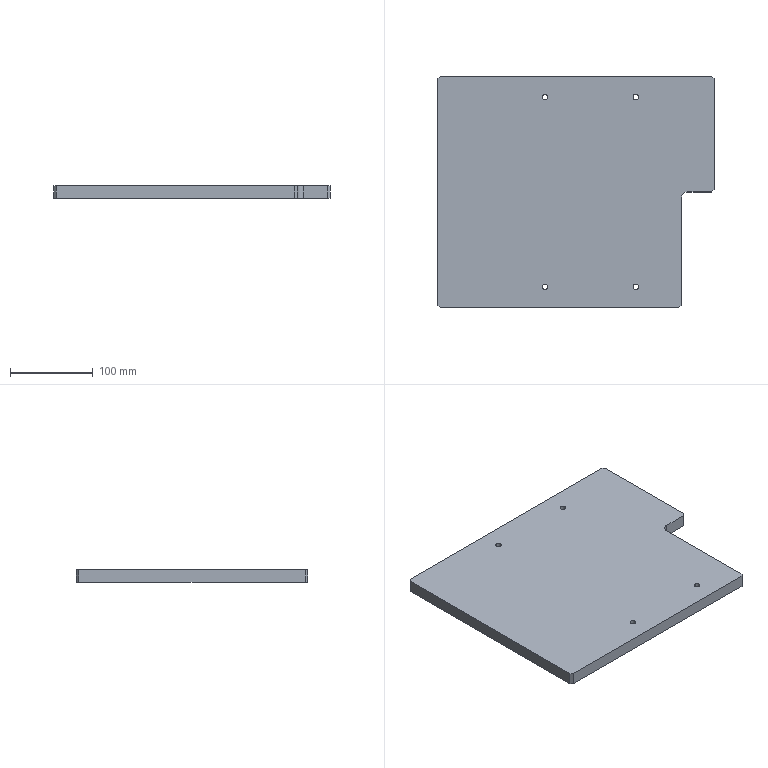Component | SolidWorks | STE21014.01-45-1 | 1 solid | 22 faces | box 335 x 280 x 15 mm | volume 1320690 mm3 | plane 13 | cylinder 9 | commonest cylinder face diameters 6.8 x8 16 x1 | material Q235
build123d program:
from build123d import *

# Parameters (mm, degrees)
SKETCH1_W           = 335
SKETCH1_H           = 280
BOSS_EXTRUDE1_DEPTH = 15
SKETCH4_W           = 40
SKETCH4_H           = 140
CUT_EXTRUDE1_DEPTH  = 219.818
M8_TAPPED_HOLE1_D   = 6.8
FILLET1_R           = 8
CHAMFER2_SIZE       = 3


with BuildPart() as part:
    # Sketch1 → Boss-Extrude1 (new body)
    with BuildSketch(Plane(origin=(0, 0, 0), x_dir=(1, 0, 0), z_dir=(0, 1, 0))):
        Rectangle(SKETCH1_W, SKETCH1_H)
    extrude(amount=BOSS_EXTRUDE1_DEPTH)

    # Sketch4 → Cut-Extrude1 (cut, through all)
    with BuildSketch(Plane(origin=(0, 15, 0), x_dir=(1, 0, 0), z_dir=(0, 1, 0))):
        with Locations((147.5, 70)):
            Rectangle(SKETCH4_W, SKETCH4_H)
    extrude(amount=-CUT_EXTRUDE1_DEPTH, mode=Mode.SUBTRACT)

    # M8 Tapped Hole1 (through all)
    with Locations(Plane(origin=(0, 15, 0), x_dir=(1, 0, 0), z_dir=(0, 1, 0))):
        with Locations((-37.5, -115), (72.5, -115), (-37.5, 115), (72.5, 115)):
            Hole(M8_TAPPED_HOLE1_D / 2)

    # Fillet1
    fillet1_edges = [part.edges().sort_by_distance(p)[0] for p in [
        (127.5, 7.5, 0),
    ]]
    fillet(fillet1_edges, radius=FILLET1_R)

    # Chamfer2
    chamfer2_edges = [part.edges().sort_by_distance(p)[0] for p in [
        (127.5, 7.5, -140),
        (167.5, 7.5, 0),
        (-167.5, 7.5, -140),
        (167.5, 7.5, 140),
        (-167.5, 7.5, 140),
    ]]
    chamfer(chamfer2_edges, length=CHAMFER2_SIZE)


solid = part.part

# Placed as in the assembly
solid = solid.moved(Location((137.5, 523.5, -90), (-90, 0, 0)))
STEP:
#1=COLOUR_RGB('',0.7922,0.8196,0.9333);
#2=FILL_AREA_STYLE_COLOUR('',#1);
#3=FILL_AREA_STYLE('',(#2));
#4=SURFACE_STYLE_FILL_AREA(#3);
#5=SURFACE_SIDE_STYLE('',(#4));
#6=SURFACE_STYLE_USAGE(.BOTH.,#5);
#7=PRESENTATION_STYLE_ASSIGNMENT((#6));
#8=CARTESIAN_POINT('',(3.937,25.004,-3.543));
#9=VERTEX_POINT('',#8);
#10=CARTESIAN_POINT('',(3.937,25.272,-3.543));
#11=VERTEX_POINT('',#10);
#12=CARTESIAN_POINT('',(3.937,25.138,-3.543));
#13=DIRECTION('',(0.,0.,-1.));
#14=DIRECTION('',(0.,1.,0.));
#15=AXIS2_PLACEMENT_3D('',#12,#13,#14);
#16=CIRCLE('',#15,0.1339);
#17=EDGE_CURVE('',#9,#11,#16,.T.);
#18=ORIENTED_EDGE('',*,*,#17,.F.);
#19=CARTESIAN_POINT('',(3.937,25.004,-4.134));
#20=VERTEX_POINT('',#19);
#21=CARTESIAN_POINT('',(3.937,25.004,-4.134));
#22=DIRECTION('',(0.,0.,-1.));
#23=VECTOR('',#22,39.37);
#24=LINE('',#21,#23);
#25=EDGE_CURVE('',#9,#20,#24,.T.);
#26=ORIENTED_EDGE('',*,*,#25,.T.);
#27=CARTESIAN_POINT('',(3.937,25.272,-4.134));
#28=VERTEX_POINT('',#27);
#29=CARTESIAN_POINT('',(3.937,25.138,-4.134));
#30=DIRECTION('',(0.,0.,-1.));
#31=DIRECTION('',(0.,1.,0.));
#32=AXIS2_PLACEMENT_3D('',#29,#30,#31);
#33=CIRCLE('',#32,0.1339);
#34=EDGE_CURVE('',#20,#28,#33,.T.);
#35=ORIENTED_EDGE('',*,*,#34,.T.);
#36=CARTESIAN_POINT('',(3.937,25.272,-4.134));
#37=DIRECTION('',(0.,0.,-1.));
#38=VECTOR('',#37,39.37);
#39=LINE('',#36,#38);
#40=EDGE_CURVE('',#11,#28,#39,.T.);
#41=ORIENTED_EDGE('',*,*,#40,.F.);
#42=EDGE_LOOP('',(#18,#26,#35,#41));
#43=FACE_OUTER_BOUND('',#42,.T.);
#44=CARTESIAN_POINT('',(3.937,25.138,-4.134));
#45=DIRECTION('',(0.,0.,-1.));
#46=DIRECTION('',(0.,1.,0.));
#47=AXIS2_PLACEMENT_3D('',#44,#45,#46);
#48=CYLINDRICAL_SURFACE('',#47,0.1339);
#49=ADVANCED_FACE('',(#43),#48,.F.);
#50=CARTESIAN_POINT('',(8.268,25.004,-3.543));
#51=VERTEX_POINT('',#50);
#52=CARTESIAN_POINT('',(8.268,25.272,-3.543));
#53=VERTEX_POINT('',#52);
#54=CARTESIAN_POINT('',(8.268,25.138,-3.543));
#55=DIRECTION('',(0.,0.,-1.));
#56=DIRECTION('',(0.,1.,0.));
#57=AXIS2_PLACEMENT_3D('',#54,#55,#56);
#58=CIRCLE('',#57,0.1339);
#59=EDGE_CURVE('',#51,#53,#58,.T.);
#60=ORIENTED_EDGE('',*,*,#59,.F.);
#61=CARTESIAN_POINT('',(8.268,25.004,-4.134));
#62=VERTEX_POINT('',#61);
#63=CARTESIAN_POINT('',(8.268,25.004,-4.134));
#64=DIRECTION('',(0.,0.,-1.));
#65=VECTOR('',#64,39.37);
#66=LINE('',#63,#65);
#67=EDGE_CURVE('',#51,#62,#66,.T.);
#68=ORIENTED_EDGE('',*,*,#67,.T.);
#69=CARTESIAN_POINT('',(8.268,25.272,-4.134));
#70=VERTEX_POINT('',#69);
#71=CARTESIAN_POINT('',(8.268,25.138,-4.134));
#72=DIRECTION('',(0.,0.,-1.));
#73=DIRECTION('',(0.,1.,0.));
#74=AXIS2_PLACEMENT_3D('',#71,#72,#73);
#75=CIRCLE('',#74,0.1339);
#76=EDGE_CURVE('',#62,#70,#75,.T.);
#77=ORIENTED_EDGE('',*,*,#76,.T.);
#78=CARTESIAN_POINT('',(8.268,25.272,-4.134));
#79=DIRECTION('',(0.,0.,-1.));
#80=VECTOR('',#79,39.37);
#81=LINE('',#78,#80);
#82=EDGE_CURVE('',#53,#70,#81,.T.);
#83=ORIENTED_EDGE('',*,*,#82,.F.);
#84=EDGE_LOOP('',(#60,#68,#77,#83));
#85=FACE_OUTER_BOUND('',#84,.T.);
#86=CARTESIAN_POINT('',(8.268,25.138,-4.134));
#87=DIRECTION('',(0.,0.,-1.));
#88=DIRECTION('',(0.,1.,0.));
#89=AXIS2_PLACEMENT_3D('',#86,#87,#88);
#90=CYLINDRICAL_SURFACE('',#89,0.1339);
#91=ADVANCED_FACE('',(#85),#90,.F.);
#92=CARTESIAN_POINT('',(3.937,15.949,-3.543));
#93=VERTEX_POINT('',#92);
#94=CARTESIAN_POINT('',(3.937,16.217,-3.543));
#95=VERTEX_POINT('',#94);
#96=CARTESIAN_POINT('',(3.937,16.083,-3.543));
#97=DIRECTION('',(0.,0.,-1.));
#98=DIRECTION('',(0.,1.,0.));
#99=AXIS2_PLACEMENT_3D('',#96,#97,#98);
#100=CIRCLE('',#99,0.1339);
#101=EDGE_CURVE('',#93,#95,#100,.T.);
#102=ORIENTED_EDGE('',*,*,#101,.F.);
#103=CARTESIAN_POINT('',(3.937,15.949,-4.134));
#104=VERTEX_POINT('',#103);
#105=CARTESIAN_POINT('',(3.937,15.949,-4.134));
#106=DIRECTION('',(0.,0.,-1.));
#107=VECTOR('',#106,39.37);
#108=LINE('',#105,#107);
#109=EDGE_CURVE('',#93,#104,#108,.T.);
#110=ORIENTED_EDGE('',*,*,#109,.T.);
#111=CARTESIAN_POINT('',(3.937,16.217,-4.134));
#112=VERTEX_POINT('',#111);
#113=CARTESIAN_POINT('',(3.937,16.083,-4.134));
#114=DIRECTION('',(0.,0.,-1.));
#115=DIRECTION('',(0.,1.,0.));
#116=AXIS2_PLACEMENT_3D('',#113,#114,#115);
#117=CIRCLE('',#116,0.1339);
#118=EDGE_CURVE('',#104,#112,#117,.T.);
#119=ORIENTED_EDGE('',*,*,#118,.T.);
#120=CARTESIAN_POINT('',(3.937,16.217,-4.134));
#121=DIRECTION('',(0.,0.,-1.));
#122=VECTOR('',#121,39.37);
#123=LINE('',#120,#122);
#124=EDGE_CURVE('',#95,#112,#123,.T.);
#125=ORIENTED_EDGE('',*,*,#124,.F.);
#126=EDGE_LOOP('',(#102,#110,#119,#125));
#127=FACE_OUTER_BOUND('',#126,.T.);
#128=CARTESIAN_POINT('',(3.937,16.083,-4.134));
#129=DIRECTION('',(0.,0.,-1.));
#130=DIRECTION('',(0.,1.,0.));
#131=AXIS2_PLACEMENT_3D('',#128,#129,#130);
#132=CYLINDRICAL_SURFACE('',#131,0.1339);
#133=ADVANCED_FACE('',(#127),#132,.F.);
#134=CARTESIAN_POINT('',(8.268,15.949,-3.543));
#135=VERTEX_POINT('',#134);
#136=CARTESIAN_POINT('',(8.268,16.217,-3.543));
#137=VERTEX_POINT('',#136);
#138=CARTESIAN_POINT('',(8.268,16.083,-3.543));
#139=DIRECTION('',(0.,0.,-1.));
#140=DIRECTION('',(0.,1.,0.));
#141=AXIS2_PLACEMENT_3D('',#138,#139,#140);
#142=CIRCLE('',#141,0.1339);
#143=EDGE_CURVE('',#135,#137,#142,.T.);
#144=ORIENTED_EDGE('',*,*,#143,.F.);
#145=CARTESIAN_POINT('',(8.268,15.949,-4.134));
#146=VERTEX_POINT('',#145);
#147=CARTESIAN_POINT('',(8.268,15.949,-4.134));
#148=DIRECTION('',(0.,0.,-1.));
#149=VECTOR('',#148,39.37);
#150=LINE('',#147,#149);
#151=EDGE_CURVE('',#135,#146,#150,.T.);
#152=ORIENTED_EDGE('',*,*,#151,.T.);
#153=CARTESIAN_POINT('',(8.268,16.217,-4.134));
#154=VERTEX_POINT('',#153);
#155=CARTESIAN_POINT('',(8.268,16.083,-4.134));
#156=DIRECTION('',(0.,0.,-1.));
#157=DIRECTION('',(0.,1.,0.));
#158=AXIS2_PLACEMENT_3D('',#155,#156,#157);
#159=CIRCLE('',#158,0.1339);
#160=EDGE_CURVE('',#146,#154,#159,.T.);
#161=ORIENTED_EDGE('',*,*,#160,.T.);
#162=CARTESIAN_POINT('',(8.268,16.217,-4.134));
#163=DIRECTION('',(0.,0.,-1.));
#164=VECTOR('',#163,39.37);
#165=LINE('',#162,#164);
#166=EDGE_CURVE('',#137,#154,#165,.T.);
#167=ORIENTED_EDGE('',*,*,#166,.F.);
#168=EDGE_LOOP('',(#144,#152,#161,#167));
#169=FACE_OUTER_BOUND('',#168,.T.);
#170=CARTESIAN_POINT('',(8.268,16.083,-4.134));
#171=DIRECTION('',(0.,0.,-1.));
#172=DIRECTION('',(0.,1.,0.));
#173=AXIS2_PLACEMENT_3D('',#170,#171,#172);
#174=CYLINDRICAL_SURFACE('',#173,0.1339);
#175=ADVANCED_FACE('',(#169),#174,.F.);
#176=CARTESIAN_POINT('',(-1.181,15.217,-4.134));
#177=VERTEX_POINT('',#176);
#178=CARTESIAN_POINT('',(-1.181,26.004,-4.134));
#179=VERTEX_POINT('',#178);
#180=CARTESIAN_POINT('',(-1.181,26.122,-4.134));
#181=DIRECTION('',(0.,1.,0.));
#182=VECTOR('',#181,39.37);
#183=LINE('',#180,#182);
#184=EDGE_CURVE('',#177,#179,#183,.T.);
#185=ORIENTED_EDGE('',*,*,#184,.F.);
#186=CARTESIAN_POINT('',(-1.181,15.217,-3.543));
#187=VERTEX_POINT('',#186);
#188=CARTESIAN_POINT('',(-1.181,15.217,-4.134));
#189=DIRECTION('',(-0.,-0.,1.));
#190=VECTOR('',#189,39.37);
#191=LINE('',#188,#190);
#192=EDGE_CURVE('',#177,#187,#191,.T.);
#193=ORIENTED_EDGE('',*,*,#192,.T.);
#194=CARTESIAN_POINT('',(-1.181,26.004,-3.543));
#195=VERTEX_POINT('',#194);
#196=CARTESIAN_POINT('',(-1.181,26.122,-3.543));
#197=DIRECTION('',(0.,1.,0.));
#198=VECTOR('',#197,39.37);
#199=LINE('',#196,#198);
#200=EDGE_CURVE('',#187,#195,#199,.T.);
#201=ORIENTED_EDGE('',*,*,#200,.T.);
#202=CARTESIAN_POINT('',(-1.181,26.004,-4.134));
#203=DIRECTION('',(0.,0.,-1.));
#204=VECTOR('',#203,39.37);
#205=LINE('',#202,#204);
#206=EDGE_CURVE('',#195,#179,#205,.T.);
#207=ORIENTED_EDGE('',*,*,#206,.T.);
#208=EDGE_LOOP('',(#185,#193,#201,#207));
#209=FACE_OUTER_BOUND('',#208,.T.);
#210=CARTESIAN_POINT('',(-1.181,26.122,-4.134));
#211=DIRECTION('',(1.,0.,-0.));
#212=DIRECTION('',(-0.,-1.,-0.));
#213=AXIS2_PLACEMENT_3D('',#210,#211,#212);
#214=PLANE('',#213);
#215=ADVANCED_FACE('',(#209),#214,.F.);
#216=CARTESIAN_POINT('',(-1.063,26.122,-4.134));
#217=VERTEX_POINT('',#216);
#218=CARTESIAN_POINT('',(11.89,26.122,-4.134));
#219=VERTEX_POINT('',#218);
#220=CARTESIAN_POINT('',(12.008,26.122,-4.134));
#221=DIRECTION('',(1.,-0.,-0.));
#222=VECTOR('',#221,39.37);
#223=LINE('',#220,#222);
#224=EDGE_CURVE('',#217,#219,#223,.T.);
#225=ORIENTED_EDGE('',*,*,#224,.F.);
#226=CARTESIAN_POINT('',(-1.063,26.122,-3.543));
#227=VERTEX_POINT('',#226);
#228=CARTESIAN_POINT('',(-1.063,26.122,-4.134));
#229=DIRECTION('',(-0.,-0.,1.));
#230=VECTOR('',#229,39.37);
#231=LINE('',#228,#230);
#232=EDGE_CURVE('',#217,#227,#231,.T.);
#233=ORIENTED_EDGE('',*,*,#232,.T.);
#234=CARTESIAN_POINT('',(11.89,26.122,-3.543));
#235=VERTEX_POINT('',#234);
#236=CARTESIAN_POINT('',(12.008,26.122,-3.543));
#237=DIRECTION('',(1.,-0.,-0.));
#238=VECTOR('',#237,39.37);
#239=LINE('',#236,#238);
#240=EDGE_CURVE('',#227,#235,#239,.T.);
#241=ORIENTED_EDGE('',*,*,#240,.T.);
#242=CARTESIAN_POINT('',(11.89,26.122,-4.134));
#243=DIRECTION('',(0.,0.,-1.));
#244=VECTOR('',#243,39.37);
#245=LINE('',#242,#244);
#246=EDGE_CURVE('',#235,#219,#245,.T.);
#247=ORIENTED_EDGE('',*,*,#246,.T.);
#248=EDGE_LOOP('',(#225,#233,#241,#247));
#249=FACE_OUTER_BOUND('',#248,.T.);
#250=CARTESIAN_POINT('',(12.008,26.122,-4.134));
#251=DIRECTION('',(-0.,-1.,-0.));
#252=DIRECTION('',(-1.,0.,0.));
#253=AXIS2_PLACEMENT_3D('',#250,#251,#252);
#254=PLANE('',#253);
#255=ADVANCED_FACE('',(#249),#254,.F.);
#256=CARTESIAN_POINT('',(12.008,26.004,-3.543));
#257=VERTEX_POINT('',#256);
#258=CARTESIAN_POINT('',(12.008,20.728,-3.543));
#259=VERTEX_POINT('',#258);
#260=CARTESIAN_POINT('',(12.008,26.122,-3.543));
#261=DIRECTION('',(-0.,-1.,-0.));
#262=VECTOR('',#261,39.37);
#263=LINE('',#260,#262);
#264=EDGE_CURVE('',#257,#259,#263,.T.);
#265=ORIENTED_EDGE('',*,*,#264,.T.);
#266=CARTESIAN_POINT('',(12.008,20.728,-4.134));
#267=VERTEX_POINT('',#266);
#268=CARTESIAN_POINT('',(12.008,20.728,-4.134));
#269=DIRECTION('',(0.,0.,-1.));
#270=VECTOR('',#269,39.37);
#271=LINE('',#268,#270);
#272=EDGE_CURVE('',#259,#267,#271,.T.);
#273=ORIENTED_EDGE('',*,*,#272,.T.);
#274=CARTESIAN_POINT('',(12.008,26.004,-4.134));
#275=VERTEX_POINT('',#274);
#276=CARTESIAN_POINT('',(12.008,26.122,-4.134));
#277=DIRECTION('',(-0.,-1.,-0.));
#278=VECTOR('',#277,39.37);
#279=LINE('',#276,#278);
#280=EDGE_CURVE('',#275,#267,#279,.T.);
#281=ORIENTED_EDGE('',*,*,#280,.F.);
#282=CARTESIAN_POINT('',(12.008,26.004,-4.134));
#283=DIRECTION('',(-0.,-0.,1.));
#284=VECTOR('',#283,39.37);
#285=LINE('',#282,#284);
#286=EDGE_CURVE('',#275,#257,#285,.T.);
#287=ORIENTED_EDGE('',*,*,#286,.T.);
#288=EDGE_LOOP('',(#265,#273,#281,#287));
#289=FACE_OUTER_BOUND('',#288,.T.);
#290=CARTESIAN_POINT('',(12.008,26.122,-4.134));
#291=DIRECTION('',(-1.,-0.,0.));
#292=DIRECTION('',(0.,1.,0.));
#293=AXIS2_PLACEMENT_3D('',#290,#291,#292);
#294=PLANE('',#293);
#295=ADVANCED_FACE('',(#289),#294,.F.);
#296=CARTESIAN_POINT('',(10.315,15.098,-3.543));
#297=VERTEX_POINT('',#296);
#298=CARTESIAN_POINT('',(-1.063,15.098,-3.543));
#299=VERTEX_POINT('',#298);
#300=CARTESIAN_POINT('',(12.008,15.098,-3.543));
#301=DIRECTION('',(-1.,0.,0.));
#302=VECTOR('',#301,39.37);
#303=LINE('',#300,#302);
#304=EDGE_CURVE('',#297,#299,#303,.T.);
#305=ORIENTED_EDGE('',*,*,#304,.T.);
#306=CARTESIAN_POINT('',(-1.063,15.098,-4.134));
#307=VERTEX_POINT('',#306);
#308=CARTESIAN_POINT('',(-1.063,15.098,-4.134));
#309=DIRECTION('',(0.,0.,-1.));
#310=VECTOR('',#309,39.37);
#311=LINE('',#308,#310);
#312=EDGE_CURVE('',#299,#307,#311,.T.);
#313=ORIENTED_EDGE('',*,*,#312,.T.);
#314=CARTESIAN_POINT('',(10.315,15.098,-4.134));
#315=VERTEX_POINT('',#314);
#316=CARTESIAN_POINT('',(12.008,15.098,-4.134));
#317=DIRECTION('',(-1.,0.,0.));
#318=VECTOR('',#317,39.37);
#319=LINE('',#316,#318);
#320=EDGE_CURVE('',#315,#307,#319,.T.);
#321=ORIENTED_EDGE('',*,*,#320,.F.);
#322=CARTESIAN_POINT('',(10.315,15.098,-4.134));
#323=DIRECTION('',(-0.,-0.,1.));
#324=VECTOR('',#323,39.37);
#325=LINE('',#322,#324);
#326=EDGE_CURVE('',#315,#297,#325,.T.);
#327=ORIENTED_EDGE('',*,*,#326,.T.);
#328=EDGE_LOOP('',(#305,#313,#321,#327));
#329=FACE_OUTER_BOUND('',#328,.T.);
#330=CARTESIAN_POINT('',(12.008,15.098,-4.134));
#331=DIRECTION('',(0.,1.,0.));
#332=DIRECTION('',(1.,-0.,-0.));
#333=AXIS2_PLACEMENT_3D('',#330,#331,#332);
#334=PLANE('',#333);
#335=ADVANCED_FACE('',(#329),#334,.F.);
#336=CARTESIAN_POINT('',(3.937,25.138,-4.134));
#337=DIRECTION('',(0.,0.,-1.));
#338=DIRECTION('',(0.,1.,0.));
#339=AXIS2_PLACEMENT_3D('',#336,#337,#338);
#340=CIRCLE('',#339,0.1339);
#341=EDGE_CURVE('',#28,#20,#340,.T.);
#342=ORIENTED_EDGE('',*,*,#341,.F.);
#343=ORIENTED_EDGE('',*,*,#34,.F.);
#344=EDGE_LOOP('',(#342,#343));
#345=FACE_BOUND('',#344,.T.);
#346=CARTESIAN_POINT('',(8.268,25.138,-4.134));
#347=DIRECTION('',(0.,0.,-1.));
#348=DIRECTION('',(0.,1.,0.));
#349=AXIS2_PLACEMENT_3D('',#346,#347,#348);
#350=CIRCLE('',#349,0.1339);
#351=EDGE_CURVE('',#70,#62,#350,.T.);
#352=ORIENTED_EDGE('',*,*,#351,.F.);
#353=ORIENTED_EDGE('',*,*,#76,.F.);
#354=EDGE_LOOP('',(#352,#353));
#355=FACE_BOUND('',#354,.T.);
#356=CARTESIAN_POINT('',(3.937,16.083,-4.134));
#357=DIRECTION('',(0.,0.,-1.));
#358=DIRECTION('',(0.,1.,0.));
#359=AXIS2_PLACEMENT_3D('',#356,#357,#358);
#360=CIRCLE('',#359,0.1339);
#361=EDGE_CURVE('',#112,#104,#360,.T.);
#362=ORIENTED_EDGE('',*,*,#361,.F.);
#363=ORIENTED_EDGE('',*,*,#118,.F.);
#364=EDGE_LOOP('',(#362,#363));
#365=FACE_BOUND('',#364,.T.);
#366=CARTESIAN_POINT('',(8.268,16.083,-4.134));
#367=DIRECTION('',(0.,0.,-1.));
#368=DIRECTION('',(0.,1.,0.));
#369=AXIS2_PLACEMENT_3D('',#366,#367,#368);
#370=CIRCLE('',#369,0.1339);
#371=EDGE_CURVE('',#154,#146,#370,.T.);
#372=ORIENTED_EDGE('',*,*,#371,.F.);
#373=ORIENTED_EDGE('',*,*,#160,.F.);
#374=EDGE_LOOP('',(#372,#373));
#375=FACE_BOUND('',#374,.T.);
#376=ORIENTED_EDGE('',*,*,#280,.T.);
#377=CARTESIAN_POINT('',(11.89,20.61,-4.134));
#378=VERTEX_POINT('',#377);
#379=CARTESIAN_POINT('',(8.652,17.372,-4.134));
#380=DIRECTION('',(-0.7071,-0.7071,0.));
#381=VECTOR('',#380,39.37);
#382=LINE('',#379,#381);
#383=EDGE_CURVE('',#267,#378,#382,.T.);
#384=ORIENTED_EDGE('',*,*,#383,.T.);
#385=CARTESIAN_POINT('',(10.748,20.61,-4.134));
#386=VERTEX_POINT('',#385);
#387=CARTESIAN_POINT('',(10.433,20.61,-4.134));
#388=DIRECTION('',(1.,-0.,-0.));
#389=VECTOR('',#388,39.37);
#390=LINE('',#387,#389);
#391=EDGE_CURVE('',#386,#378,#390,.T.);
#392=ORIENTED_EDGE('',*,*,#391,.F.);
#393=CARTESIAN_POINT('',(10.433,20.295,-4.134));
#394=VERTEX_POINT('',#393);
#395=CARTESIAN_POINT('',(10.748,20.295,-4.134));
#396=DIRECTION('',(-0.,-0.,1.));
#397=DIRECTION('',(0.,1.,0.));
#398=AXIS2_PLACEMENT_3D('',#395,#396,#397);
#399=CIRCLE('',#398,0.315);
#400=EDGE_CURVE('',#386,#394,#399,.T.);
#401=ORIENTED_EDGE('',*,*,#400,.T.);
#402=CARTESIAN_POINT('',(10.433,15.217,-4.134));
#403=VERTEX_POINT('',#402);
#404=CARTESIAN_POINT('',(10.433,20.61,-4.134));
#405=DIRECTION('',(0.,1.,0.));
#406=VECTOR('',#405,39.37);
#407=LINE('',#404,#406);
#408=EDGE_CURVE('',#403,#394,#407,.T.);
#409=ORIENTED_EDGE('',*,*,#408,.F.);
#410=CARTESIAN_POINT('',(10.62,15.404,-4.134));
#411=DIRECTION('',(-0.7071,-0.7071,0.));
#412=VECTOR('',#411,39.37);
#413=LINE('',#410,#412);
#414=EDGE_CURVE('',#403,#315,#413,.T.);
#415=ORIENTED_EDGE('',*,*,#414,.T.);
#416=ORIENTED_EDGE('',*,*,#320,.T.);
#417=CARTESIAN_POINT('',(-0.5807,14.616,-4.134));
#418=DIRECTION('',(-0.7071,0.7071,0.));
#419=VECTOR('',#418,39.37);
#420=LINE('',#417,#419);
#421=EDGE_CURVE('',#307,#177,#420,.T.);
#422=ORIENTED_EDGE('',*,*,#421,.T.);
#423=ORIENTED_EDGE('',*,*,#184,.T.);
#424=CARTESIAN_POINT('',(-0.5807,26.604,-4.134));
#425=DIRECTION('',(0.7071,0.7071,-0.));
#426=VECTOR('',#425,39.37);
#427=LINE('',#424,#426);
#428=EDGE_CURVE('',#179,#217,#427,.T.);
#429=ORIENTED_EDGE('',*,*,#428,.T.);
#430=ORIENTED_EDGE('',*,*,#224,.T.);
#431=CARTESIAN_POINT('',(11.407,26.604,-4.134));
#432=DIRECTION('',(0.7071,-0.7071,-0.));
#433=VECTOR('',#432,39.37);
#434=LINE('',#431,#433);
#435=EDGE_CURVE('',#219,#275,#434,.T.);
#436=ORIENTED_EDGE('',*,*,#435,.T.);
#437=EDGE_LOOP('',(#376,#384,#392,#401,#409,#415,#416,#422,#423,#429,#430,#436));
#438=FACE_OUTER_BOUND('',#437,.T.);
#439=CARTESIAN_POINT('',(5.413,20.61,-4.134));
#440=DIRECTION('',(0.,0.,-1.));
#441=DIRECTION('',(0.,1.,0.));
#442=AXIS2_PLACEMENT_3D('',#439,#440,#441);
#443=PLANE('',#442);
#444=ADVANCED_FACE('',(#345,#355,#365,#375,#438),#443,.T.);
#445=CARTESIAN_POINT('',(3.937,25.138,-3.543));
#446=DIRECTION('',(0.,0.,-1.));
#447=DIRECTION('',(0.,1.,0.));
#448=AXIS2_PLACEMENT_3D('',#445,#446,#447);
#449=CIRCLE('',#448,0.1339);
#450=EDGE_CURVE('',#11,#9,#449,.T.);
#451=ORIENTED_EDGE('',*,*,#450,.T.);
#452=ORIENTED_EDGE('',*,*,#17,.T.);
#453=EDGE_LOOP('',(#451,#452));
#454=FACE_BOUND('',#453,.T.);
#455=CARTESIAN_POINT('',(8.268,25.138,-3.543));
#456=DIRECTION('',(0.,0.,-1.));
#457=DIRECTION('',(0.,1.,0.));
#458=AXIS2_PLACEMENT_3D('',#455,#456,#457);
#459=CIRCLE('',#458,0.1339);
#460=EDGE_CURVE('',#53,#51,#459,.T.);
#461=ORIENTED_EDGE('',*,*,#460,.T.);
#462=ORIENTED_EDGE('',*,*,#59,.T.);
#463=EDGE_LOOP('',(#461,#462));
#464=FACE_BOUND('',#463,.T.);
#465=CARTESIAN_POINT('',(3.937,16.083,-3.543));
#466=DIRECTION('',(0.,0.,-1.));
#467=DIRECTION('',(0.,1.,0.));
#468=AXIS2_PLACEMENT_3D('',#465,#466,#467);
#469=CIRCLE('',#468,0.1339);
#470=EDGE_CURVE('',#95,#93,#469,.T.);
#471=ORIENTED_EDGE('',*,*,#470,.T.);
#472=ORIENTED_EDGE('',*,*,#101,.T.);
#473=EDGE_LOOP('',(#471,#472));
#474=FACE_BOUND('',#473,.T.);
#475=CARTESIAN_POINT('',(8.268,16.083,-3.543));
#476=DIRECTION('',(0.,0.,-1.));
#477=DIRECTION('',(0.,1.,0.));
#478=AXIS2_PLACEMENT_3D('',#475,#476,#477);
#479=CIRCLE('',#478,0.1339);
#480=EDGE_CURVE('',#137,#135,#479,.T.);
#481=ORIENTED_EDGE('',*,*,#480,.T.);
#482=ORIENTED_EDGE('',*,*,#143,.T.);
#483=EDGE_LOOP('',(#481,#482));
#484=FACE_BOUND('',#483,.T.);
#485=CARTESIAN_POINT('',(10.748,20.61,-3.543));
#486=VERTEX_POINT('',#485);
#487=CARTESIAN_POINT('',(11.89,20.61,-3.543));
#488=VERTEX_POINT('',#487);
#489=CARTESIAN_POINT('',(10.433,20.61,-3.543));
#490=DIRECTION('',(1.,-0.,-0.));
#491=VECTOR('',#490,39.37);
#492=LINE('',#489,#491);
#493=EDGE_CURVE('',#486,#488,#492,.T.);
#494=ORIENTED_EDGE('',*,*,#493,.T.);
#495=CARTESIAN_POINT('',(12.008,20.728,-3.543));
#496=DIRECTION('',(0.7071,0.7071,-0.));
#497=VECTOR('',#496,39.37);
#498=LINE('',#495,#497);
#499=EDGE_CURVE('',#488,#259,#498,.T.);
#500=ORIENTED_EDGE('',*,*,#499,.T.);
#501=ORIENTED_EDGE('',*,*,#264,.F.);
#502=CARTESIAN_POINT('',(12.008,26.004,-3.543));
#503=DIRECTION('',(-0.7071,0.7071,0.));
#504=VECTOR('',#503,39.37);
#505=LINE('',#502,#504);
#506=EDGE_CURVE('',#257,#235,#505,.T.);
#507=ORIENTED_EDGE('',*,*,#506,.T.);
#508=ORIENTED_EDGE('',*,*,#240,.F.);
#509=CARTESIAN_POINT('',(-1.063,26.122,-3.543));
#510=DIRECTION('',(-0.7071,-0.7071,0.));
#511=VECTOR('',#510,39.37);
#512=LINE('',#509,#511);
#513=EDGE_CURVE('',#227,#195,#512,.T.);
#514=ORIENTED_EDGE('',*,*,#513,.T.);
#515=ORIENTED_EDGE('',*,*,#200,.F.);
#516=CARTESIAN_POINT('',(-1.181,15.217,-3.543));
#517=DIRECTION('',(0.7071,-0.7071,-0.));
#518=VECTOR('',#517,39.37);
#519=LINE('',#516,#518);
#520=EDGE_CURVE('',#187,#299,#519,.T.);
#521=ORIENTED_EDGE('',*,*,#520,.T.);
#522=ORIENTED_EDGE('',*,*,#304,.F.);
#523=CARTESIAN_POINT('',(10.433,15.217,-3.543));
#524=VERTEX_POINT('',#523);
#525=CARTESIAN_POINT('',(10.433,15.217,-3.543));
#526=DIRECTION('',(0.7071,0.7071,-0.));
#527=VECTOR('',#526,39.37);
#528=LINE('',#525,#527);
#529=EDGE_CURVE('',#297,#524,#528,.T.);
#530=ORIENTED_EDGE('',*,*,#529,.T.);
#531=CARTESIAN_POINT('',(10.433,20.295,-3.543));
#532=VERTEX_POINT('',#531);
#533=CARTESIAN_POINT('',(10.433,20.61,-3.543));
#534=DIRECTION('',(0.,1.,0.));
#535=VECTOR('',#534,39.37);
#536=LINE('',#533,#535);
#537=EDGE_CURVE('',#524,#532,#536,.T.);
#538=ORIENTED_EDGE('',*,*,#537,.T.);
#539=CARTESIAN_POINT('',(10.748,20.295,-3.543));
#540=DIRECTION('',(0.,0.,-1.));
#541=DIRECTION('',(0.,1.,0.));
#542=AXIS2_PLACEMENT_3D('',#539,#540,#541);
#543=CIRCLE('',#542,0.315);
#544=EDGE_CURVE('',#532,#486,#543,.T.);
#545=ORIENTED_EDGE('',*,*,#544,.T.);
#546=EDGE_LOOP('',(#494,#500,#501,#507,#508,#514,#515,#521,#522,#530,#538,#545));
#547=FACE_OUTER_BOUND('',#546,.T.);
#548=CARTESIAN_POINT('',(5.413,20.61,-3.543));
#549=DIRECTION('',(0.,0.,-1.));
#550=DIRECTION('',(0.,1.,0.));
#551=AXIS2_PLACEMENT_3D('',#548,#549,#550);
#552=PLANE('',#551);
#553=ADVANCED_FACE('',(#454,#464,#474,#484,#547),#552,.F.);
#554=ORIENTED_EDGE('',*,*,#537,.F.);
#555=CARTESIAN_POINT('',(10.433,15.217,-3.543));
#556=DIRECTION('',(0.,0.,-1.));
#557=VECTOR('',#556,39.37);
#558=LINE('',#555,#557);
#559=EDGE_CURVE('',#524,#403,#558,.T.);
#560=ORIENTED_EDGE('',*,*,#559,.T.);
#561=ORIENTED_EDGE('',*,*,#408,.T.);
#562=CARTESIAN_POINT('',(10.433,20.295,-3.543));
#563=DIRECTION('',(-0.,-0.,1.));
#564=VECTOR('',#563,39.37);
#565=LINE('',#562,#564);
#566=EDGE_CURVE('',#394,#532,#565,.T.);
#567=ORIENTED_EDGE('',*,*,#566,.T.);
#568=EDGE_LOOP('',(#554,#560,#561,#567));
#569=FACE_OUTER_BOUND('',#568,.T.);
#570=CARTESIAN_POINT('',(10.433,20.61,-3.543));
#571=DIRECTION('',(-1.,-0.,0.));
#572=DIRECTION('',(0.,1.,0.));
#573=AXIS2_PLACEMENT_3D('',#570,#571,#572);
#574=PLANE('',#573);
#575=ADVANCED_FACE('',(#569),#574,.F.);
#576=ORIENTED_EDGE('',*,*,#391,.T.);
#577=CARTESIAN_POINT('',(11.89,20.61,-3.543));
#578=DIRECTION('',(-0.,-0.,1.));
#579=VECTOR('',#578,39.37);
#580=LINE('',#577,#579);
#581=EDGE_CURVE('',#378,#488,#580,.T.);
#582=ORIENTED_EDGE('',*,*,#581,.T.);
#583=ORIENTED_EDGE('',*,*,#493,.F.);
#584=CARTESIAN_POINT('',(10.748,20.61,-4.134));
#585=DIRECTION('',(0.,0.,-1.));
#586=VECTOR('',#585,39.37);
#587=LINE('',#584,#586);
#588=EDGE_CURVE('',#486,#386,#587,.T.);
#589=ORIENTED_EDGE('',*,*,#588,.T.);
#590=EDGE_LOOP('',(#576,#582,#583,#589));
#591=FACE_OUTER_BOUND('',#590,.T.);
#592=CARTESIAN_POINT('',(10.433,20.61,-3.543));
#593=DIRECTION('',(0.,1.,0.));
#594=DIRECTION('',(1.,-0.,-0.));
#595=AXIS2_PLACEMENT_3D('',#592,#593,#594);
#596=PLANE('',#595);
#597=ADVANCED_FACE('',(#591),#596,.F.);
#598=ORIENTED_EDGE('',*,*,#151,.F.);
#599=ORIENTED_EDGE('',*,*,#480,.F.);
#600=ORIENTED_EDGE('',*,*,#166,.T.);
#601=ORIENTED_EDGE('',*,*,#371,.T.);
#602=EDGE_LOOP('',(#598,#599,#600,#601));
#603=FACE_OUTER_BOUND('',#602,.T.);
#604=CARTESIAN_POINT('',(8.268,16.083,-4.134));
#605=DIRECTION('',(0.,0.,-1.));
#606=DIRECTION('',(0.,1.,0.));
#607=AXIS2_PLACEMENT_3D('',#604,#605,#606);
#608=CYLINDRICAL_SURFACE('',#607,0.1339);
#609=ADVANCED_FACE('',(#603),#608,.F.);
#610=ORIENTED_EDGE('',*,*,#109,.F.);
#611=ORIENTED_EDGE('',*,*,#470,.F.);
#612=ORIENTED_EDGE('',*,*,#124,.T.);
#613=ORIENTED_EDGE('',*,*,#361,.T.);
#614=EDGE_LOOP('',(#610,#611,#612,#613));
#615=FACE_OUTER_BOUND('',#614,.T.);
#616=CARTESIAN_POINT('',(3.937,16.083,-4.134));
#617=DIRECTION('',(0.,0.,-1.));
#618=DIRECTION('',(0.,1.,0.));
#619=AXIS2_PLACEMENT_3D('',#616,#617,#618);
#620=CYLINDRICAL_SURFACE('',#619,0.1339);
#621=ADVANCED_FACE('',(#615),#620,.F.);
#622=ORIENTED_EDGE('',*,*,#67,.F.);
#623=ORIENTED_EDGE('',*,*,#460,.F.);
#624=ORIENTED_EDGE('',*,*,#82,.T.);
#625=ORIENTED_EDGE('',*,*,#351,.T.);
#626=EDGE_LOOP('',(#622,#623,#624,#625));
#627=FACE_OUTER_BOUND('',#626,.T.);
#628=CARTESIAN_POINT('',(8.268,25.138,-4.134));
#629=DIRECTION('',(0.,0.,-1.));
#630=DIRECTION('',(0.,1.,0.));
#631=AXIS2_PLACEMENT_3D('',#628,#629,#630);
#632=CYLINDRICAL_SURFACE('',#631,0.1339);
#633=ADVANCED_FACE('',(#627),#632,.F.);
#634=ORIENTED_EDGE('',*,*,#25,.F.);
#635=ORIENTED_EDGE('',*,*,#450,.F.);
#636=ORIENTED_EDGE('',*,*,#40,.T.);
#637=ORIENTED_EDGE('',*,*,#341,.T.);
#638=EDGE_LOOP('',(#634,#635,#636,#637));
#639=FACE_OUTER_BOUND('',#638,.T.);
#640=CARTESIAN_POINT('',(3.937,25.138,-4.134));
#641=DIRECTION('',(0.,0.,-1.));
#642=DIRECTION('',(0.,1.,0.));
#643=AXIS2_PLACEMENT_3D('',#640,#641,#642);
#644=CYLINDRICAL_SURFACE('',#643,0.1339);
#645=ADVANCED_FACE('',(#639),#644,.F.);
#646=ORIENTED_EDGE('',*,*,#544,.F.);
#647=ORIENTED_EDGE('',*,*,#566,.F.);
#648=ORIENTED_EDGE('',*,*,#400,.F.);
#649=ORIENTED_EDGE('',*,*,#588,.F.);
#650=EDGE_LOOP('',(#646,#647,#648,#649));
#651=FACE_OUTER_BOUND('',#650,.T.);
#652=CARTESIAN_POINT('',(10.748,20.295,-3.543));
#653=DIRECTION('',(-0.,-0.,1.));
#654=DIRECTION('',(0.,-1.,0.));
#655=AXIS2_PLACEMENT_3D('',#652,#653,#654);
#656=CYLINDRICAL_SURFACE('',#655,0.315);
#657=ADVANCED_FACE('',(#651),#656,.F.);
#658=ORIENTED_EDGE('',*,*,#499,.F.);
#659=ORIENTED_EDGE('',*,*,#581,.F.);
#660=ORIENTED_EDGE('',*,*,#383,.F.);
#661=ORIENTED_EDGE('',*,*,#272,.F.);
#662=EDGE_LOOP('',(#658,#659,#660,#661));
#663=FACE_OUTER_BOUND('',#662,.T.);
#664=CARTESIAN_POINT('',(12.008,20.728,-4.134));
#665=DIRECTION('',(-0.7071,0.7071,0.));
#666=DIRECTION('',(0.,0.,-1.));
#667=AXIS2_PLACEMENT_3D('',#664,#665,#666);
#668=PLANE('',#667);
#669=ADVANCED_FACE('',(#663),#668,.F.);
#670=ORIENTED_EDGE('',*,*,#421,.F.);
#671=ORIENTED_EDGE('',*,*,#312,.F.);
#672=ORIENTED_EDGE('',*,*,#520,.F.);
#673=ORIENTED_EDGE('',*,*,#192,.F.);
#674=EDGE_LOOP('',(#670,#671,#672,#673));
#675=FACE_OUTER_BOUND('',#674,.T.);
#676=CARTESIAN_POINT('',(-1.181,15.217,-4.134));
#677=DIRECTION('',(0.7071,0.7071,0.));
#678=DIRECTION('',(-0.,-0.,1.));
#679=AXIS2_PLACEMENT_3D('',#676,#677,#678);
#680=PLANE('',#679);
#681=ADVANCED_FACE('',(#675),#680,.F.);
#682=ORIENTED_EDGE('',*,*,#428,.F.);
#683=ORIENTED_EDGE('',*,*,#206,.F.);
#684=ORIENTED_EDGE('',*,*,#513,.F.);
#685=ORIENTED_EDGE('',*,*,#232,.F.);
#686=EDGE_LOOP('',(#682,#683,#684,#685));
#687=FACE_OUTER_BOUND('',#686,.T.);
#688=CARTESIAN_POINT('',(-1.063,26.122,-4.134));
#689=DIRECTION('',(0.7071,-0.7071,-0.));
#690=DIRECTION('',(-0.,-0.,1.));
#691=AXIS2_PLACEMENT_3D('',#688,#689,#690);
#692=PLANE('',#691);
#693=ADVANCED_FACE('',(#687),#692,.F.);
#694=ORIENTED_EDGE('',*,*,#435,.F.);
#695=ORIENTED_EDGE('',*,*,#246,.F.);
#696=ORIENTED_EDGE('',*,*,#506,.F.);
#697=ORIENTED_EDGE('',*,*,#286,.F.);
#698=EDGE_LOOP('',(#694,#695,#696,#697));
#699=FACE_OUTER_BOUND('',#698,.T.);
#700=CARTESIAN_POINT('',(12.008,26.004,-4.134));
#701=DIRECTION('',(-0.7071,-0.7071,-0.));
#702=DIRECTION('',(-0.,-0.,1.));
#703=AXIS2_PLACEMENT_3D('',#700,#701,#702);
#704=PLANE('',#703);
#705=ADVANCED_FACE('',(#699),#704,.F.);
#706=ORIENTED_EDGE('',*,*,#529,.F.);
#707=ORIENTED_EDGE('',*,*,#326,.F.);
#708=ORIENTED_EDGE('',*,*,#414,.F.);
#709=ORIENTED_EDGE('',*,*,#559,.F.);
#710=EDGE_LOOP('',(#706,#707,#708,#709));
#711=FACE_OUTER_BOUND('',#710,.T.);
#712=CARTESIAN_POINT('',(10.433,15.217,-3.543));
#713=DIRECTION('',(-0.7071,0.7071,0.));
#714=DIRECTION('',(0.,0.,-1.));
#715=AXIS2_PLACEMENT_3D('',#712,#713,#714);
#716=PLANE('',#715);
#717=ADVANCED_FACE('',(#711),#716,.F.);
#718=CLOSED_SHELL('',(#49,#91,#133,#175,#215,#255,#295,#335,#444,#553,#575,#597,#609,#621,#633,#645,#657,#669,#681,#693,#705,#717));
#719=MANIFOLD_SOLID_BREP('',#718);
#720=STYLED_ITEM('',(#7),#719);
#721=(LENGTH_UNIT()NAMED_UNIT(*)SI_UNIT($,.METRE.));
#722=LENGTH_MEASURE_WITH_UNIT(LENGTH_MEASURE(0.0254),#721);
#723=DIMENSIONAL_EXPONENTS(1.,0.,0.,0.,0.,0.,0.);
#724=(CONVERSION_BASED_UNIT('',#722)LENGTH_UNIT()NAMED_UNIT(#723));
#725=UNCERTAINTY_MEASURE_WITH_UNIT(LENGTH_MEASURE(0.00001),#724,'','');
#726=(NAMED_UNIT(*)PLANE_ANGLE_UNIT()SI_UNIT($,.RADIAN.));
#727=(NAMED_UNIT(*)SI_UNIT($,.STERADIAN.)SOLID_ANGLE_UNIT());
#728=(GEOMETRIC_REPRESENTATION_CONTEXT(3)GLOBAL_UNCERTAINTY_ASSIGNED_CONTEXT((#725))GLOBAL_UNIT_ASSIGNED_CONTEXT((#724,#726,#727))REPRESENTATION_CONTEXT('',''));
#729=MECHANICAL_DESIGN_GEOMETRIC_PRESENTATION_REPRESENTATION('',(#720),#728);
#730=CARTESIAN_POINT('',(0.,0.,0.));
#731=DIRECTION('',(0.,0.,1.));
#732=DIRECTION('',(1.,0.,0.));
#733=AXIS2_PLACEMENT_3D('',#730,#731,#732);
#734=(LENGTH_UNIT()NAMED_UNIT(*)SI_UNIT($,.METRE.));
#735=LENGTH_MEASURE_WITH_UNIT(LENGTH_MEASURE(0.0254),#734);
#736=DIMENSIONAL_EXPONENTS(1.,0.,0.,0.,0.,0.,0.);
#737=(CONVERSION_BASED_UNIT('',#735)LENGTH_UNIT()NAMED_UNIT(#736));
#738=UNCERTAINTY_MEASURE_WITH_UNIT(LENGTH_MEASURE(0.00001),#737,'','');
#739=(NAMED_UNIT(*)PLANE_ANGLE_UNIT()SI_UNIT($,.RADIAN.));
#740=(NAMED_UNIT(*)SI_UNIT($,.STERADIAN.)SOLID_ANGLE_UNIT());
#741=(GEOMETRIC_REPRESENTATION_CONTEXT(3)GLOBAL_UNCERTAINTY_ASSIGNED_CONTEXT((#738))GLOBAL_UNIT_ASSIGNED_CONTEXT((#737,#739,#740))REPRESENTATION_CONTEXT('',''));
#742=ADVANCED_BREP_SHAPE_REPRESENTATION('',(#719,#733),#741);
#743=PRESENTATION_LAYER_ASSIGNMENT('','',(#720));